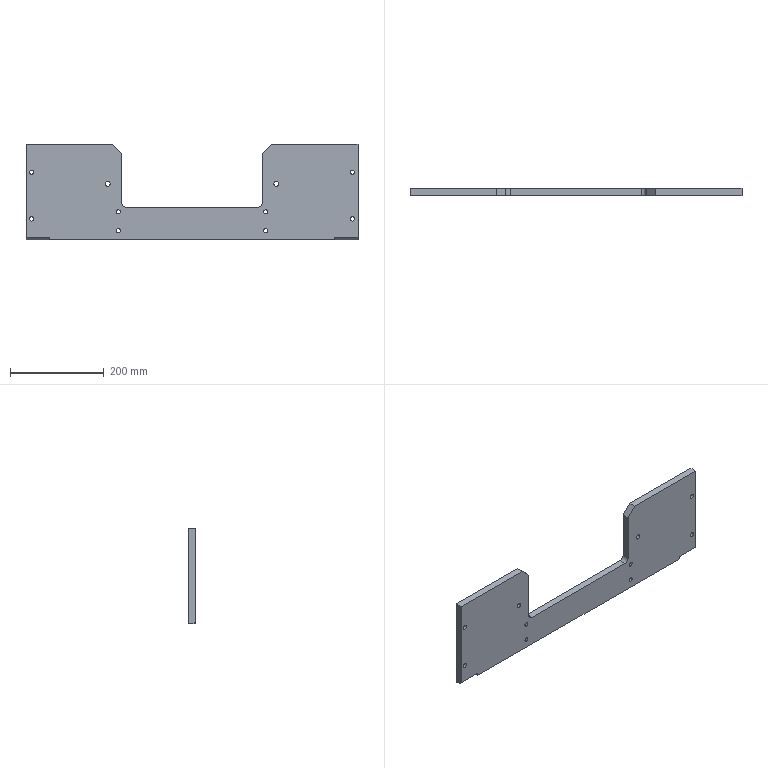Component | SolidWorks | FrameAssembly-1_FormerSupportPlate-1 | 1 solid | 66 faces | box 709 x 15 x 205 mm | volume 1550833 mm3 | cylinder 38 | plane 24 | cone 4 | commonest cylinder face diameters 9 x16 13 x8 14 x8 10.2 x4 20 x2
build123d program:
from build123d import *

# Parameters (mm, degrees)
SKETCH1_W                                            = 709
SKETCH1_H                                            = 205
BOSS_EXTRUDE1_DEPTH                                  = 15
SKETCH2_W                                            = 300
SKETCH2_H                                            = 135
CUT_EXTRUDE1_DEPTH                                   = 410.781
CUT_EXTRUDE2_DEPTH                                   = 50
CUT_EXTRUDE3_DEPTH                                   = 50
F_10_2_10_2_DIAMETER_HOLE1_D                         = 10.2
CYLINDRICAL_COUNTERSUNK_HOLE_1_FOR_M8_HE_D           = 9
CYLINDRICAL_COUNTERSUNK_HOLE_1_FOR_M8_HE_CBORE_D     = 14
CYLINDRICAL_COUNTERSUNK_HOLE_1_FOR_M8_HE_CBORE_DEPTH = 5
CYLINDRICAL_COUNTERSUNK_HOLE_2_FOR_M8_HE_D           = 9
CYLINDRICAL_COUNTERSUNK_HOLE_2_FOR_M8_HE_CBORE_D     = 13
CYLINDRICAL_COUNTERSUNK_HOLE_2_FOR_M8_HE_CBORE_DEPTH = 10
CHAMFER1_SIZE                                        = 20
CHAMFER2_SIZE                                        = 0.925
FILLET1_R                                            = 10


with BuildPart() as part:
    # Sketch1 → Boss-Extrude1 (new body)
    with BuildSketch(Plane.XY.offset(7.5)):
        with Locations((0, -102.5)):
            Rectangle(SKETCH1_W, SKETCH1_H)
    extrude(amount=-BOSS_EXTRUDE1_DEPTH)

    # Sketch2 → Cut-Extrude1 (cut, through all)
    with BuildSketch(Plane(origin=(0, 0, -7.5), x_dir=(-1, 0, 0), z_dir=(0, 0, -1))):
        with Locations((0, -137.5)):
            Rectangle(SKETCH2_W, SKETCH2_H)
    extrude(amount=-CUT_EXTRUDE1_DEPTH, mode=Mode.SUBTRACT)

    # Sketch3 → Cut-Extrude2 (cut)
    with BuildSketch(Plane(origin=(354.5, 0, 0), x_dir=(0, 0, -1), z_dir=(1, 0, 0))):
        Polygon((1.5, 0), (7.5, -6), (7.5, 0), align=None)
    extrude(amount=-CUT_EXTRUDE2_DEPTH, mode=Mode.SUBTRACT)

    # Sketch4 → Cut-Extrude3 (cut)
    with BuildSketch(Plane.ZY.offset(354.5)):
        Polygon((-7.5, 0), (-7.5, -6), (-1.5, 0), align=None)
    extrude(amount=-CUT_EXTRUDE3_DEPTH, mode=Mode.SUBTRACT)

    # 10.2 _10.2_ Diameter Hole1 (through all)
    with Locations(Plane.XY.offset(7.5)):
        with Locations((-180, -120), (180, -120)):
            Hole(F_10_2_10_2_DIAMETER_HOLE1_D / 2)

    # Cylindrical Countersunk Hole 1 for M8 He (through all)
    with Locations(Plane.XY.offset(7.5)):
        with Locations((342.5, -145), (-342.5, -45), (-342.5, -145), (342.5, -45)):
            CounterBoreHole(CYLINDRICAL_COUNTERSUNK_HOLE_1_FOR_M8_HE_D / 2, CYLINDRICAL_COUNTERSUNK_HOLE_1_FOR_M8_HE_CBORE_D / 2, CYLINDRICAL_COUNTERSUNK_HOLE_1_FOR_M8_HE_CBORE_DEPTH)

    # Cylindrical Countersunk Hole 2 for M8 He (through all)
    with Locations(Plane.XY.offset(7.5)):
        with Locations((-157.5, -60), (157.5, -60), (157.5, -20), (-157.5, -20)):
            CounterBoreHole(CYLINDRICAL_COUNTERSUNK_HOLE_2_FOR_M8_HE_D / 2, CYLINDRICAL_COUNTERSUNK_HOLE_2_FOR_M8_HE_CBORE_D / 2, CYLINDRICAL_COUNTERSUNK_HOLE_2_FOR_M8_HE_CBORE_DEPTH)

    # Chamfer1
    chamfer1_edges = [part.edges().sort_by_distance(p)[0] for p in [
        (-150, -205, 0),
        (150, -205, 0),
    ]]
    chamfer(chamfer1_edges, length=CHAMFER1_SIZE)

    # Chamfer2
    chamfer2_edges = [part.edges().sort_by_distance(p)[0] for p in [
        (185.1, -120, 7.5),
        (-174.9, -120, 7.5),
    ]]
    chamfer(chamfer2_edges, length=CHAMFER2_SIZE)

    # Fillet1
    fillet1_edges = [part.edges().sort_by_distance(p)[0] for p in [
        (150, -70, 0),
        (-150, -70, 0),
    ]]
    fillet(fillet1_edges, radius=FILLET1_R)


solid = part.part

# Placed as in the assembly
solid = solid.moved(Location((-298.746, 368.873, -16.5), (-90, 0, 0)))